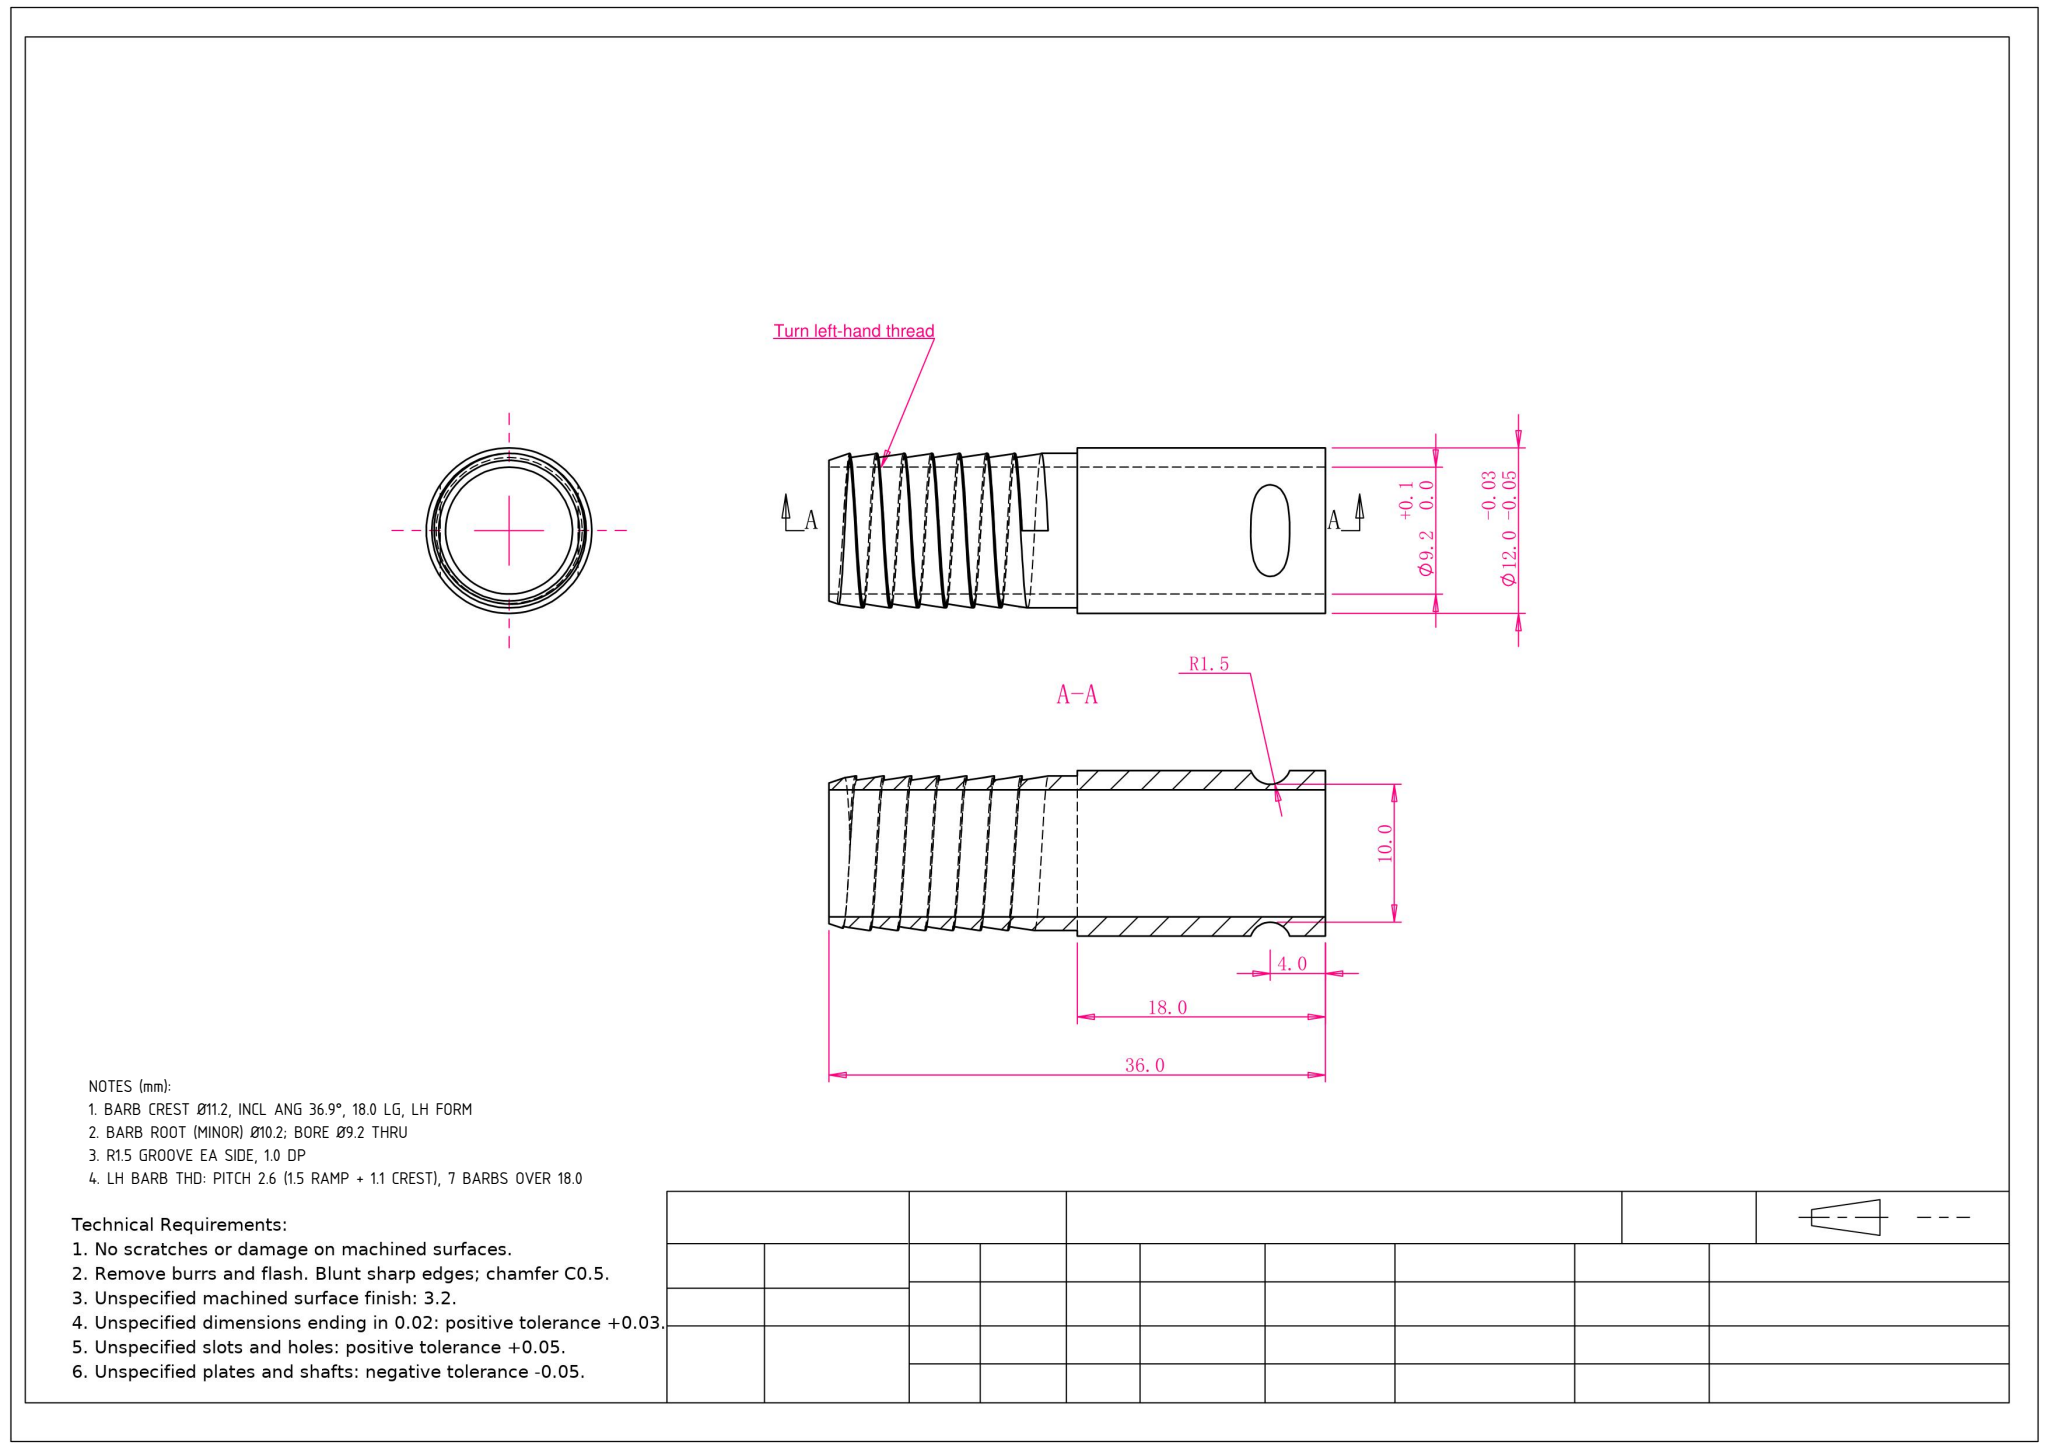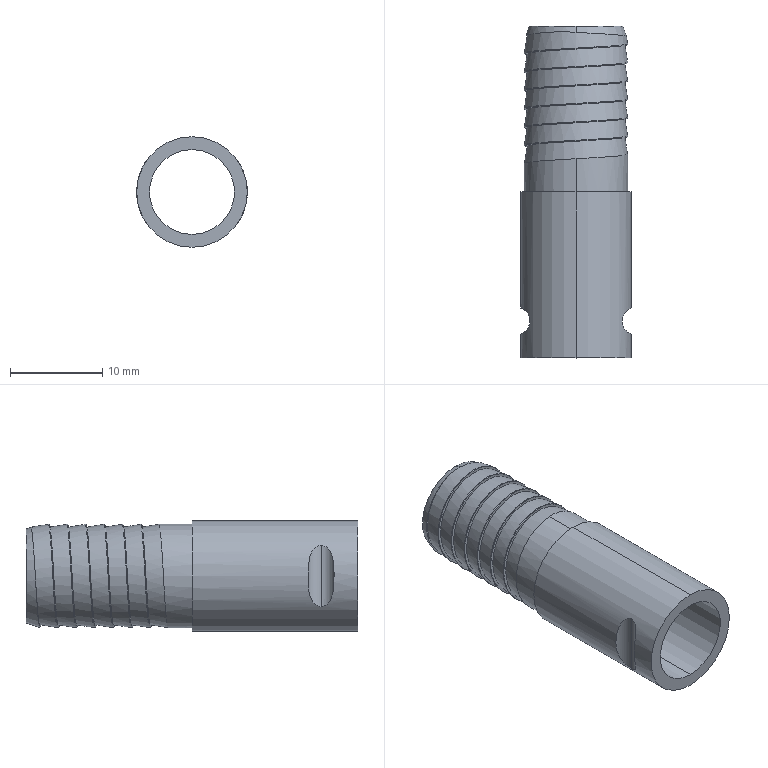Part | SolidWorks | mm | 1 solid | 29 faces | box 12 x 36 x 12 mm | volume 1321 mm3 | cylinder 21 | plane 4 | cone 2 | spline 2 | commonest cylinder face diameters 11.2 x14 3 x3 9.2 x2 12 x2
Drawing notes:
BARB CREST Ø11.2, INCL ANG 36.9°, 18.0 LG, LH FORM | from the solid: cyls dia 11.2 axis y (crests); cones incl ang 36.9; barbed section 18.0 of 36.0 OAL
BARB ROOT (MINOR) Ø10.2; BORE Ø9.2 THRU | from the solid: cones ref_dia 10.2 at taper start; cyl dia 9.2 axis y, length 36.0 thru
R1.5 GROOVE EA SIDE, 1.0 DP | from the solid: Ø3.0 cutter cyls axis z at x=-0.5 and x=12.5 on Ø12 shaft (x 0..12) = 1.0 deep each side
LH BARB THD: PITCH 2.6 (1.5 RAMP + 1.1 CREST), 7 BARBS OVER 18.0 | from the solid: cones 36.9deg from Ø10.2 root to Ø11.2 crest = 1.5 axial ramp; Ø11.2 crest faces 1.1 long (11x) => 2.6 pitch; 14 crest faces = 7 turns x 2 over 18.0 barb length (Ø12.0 shank 18.0 of 36.0 total)